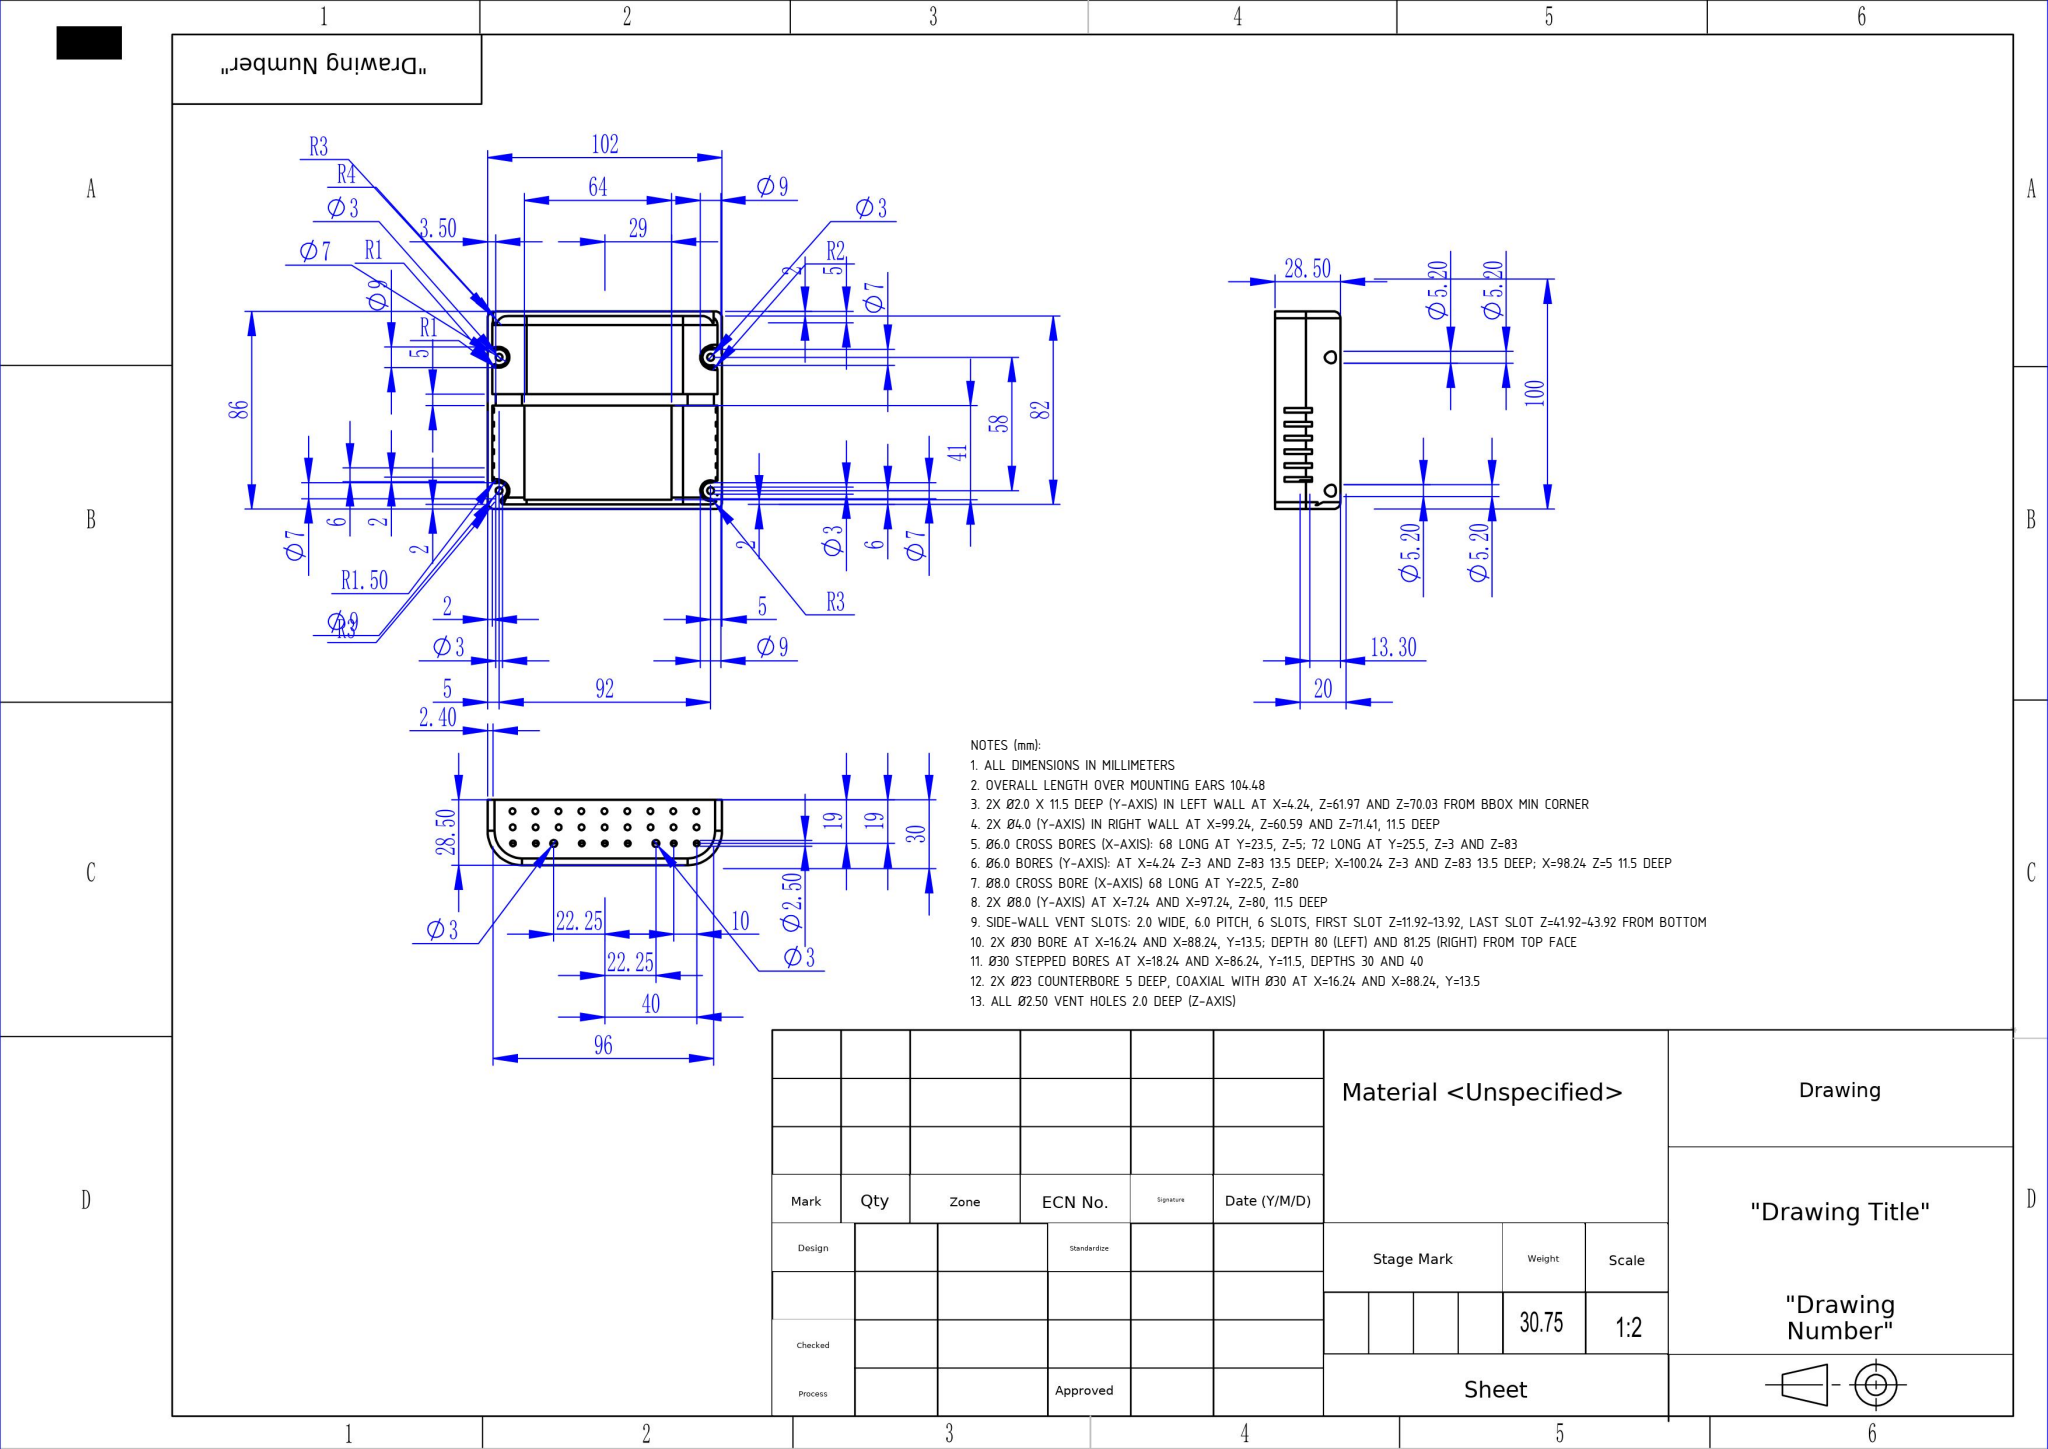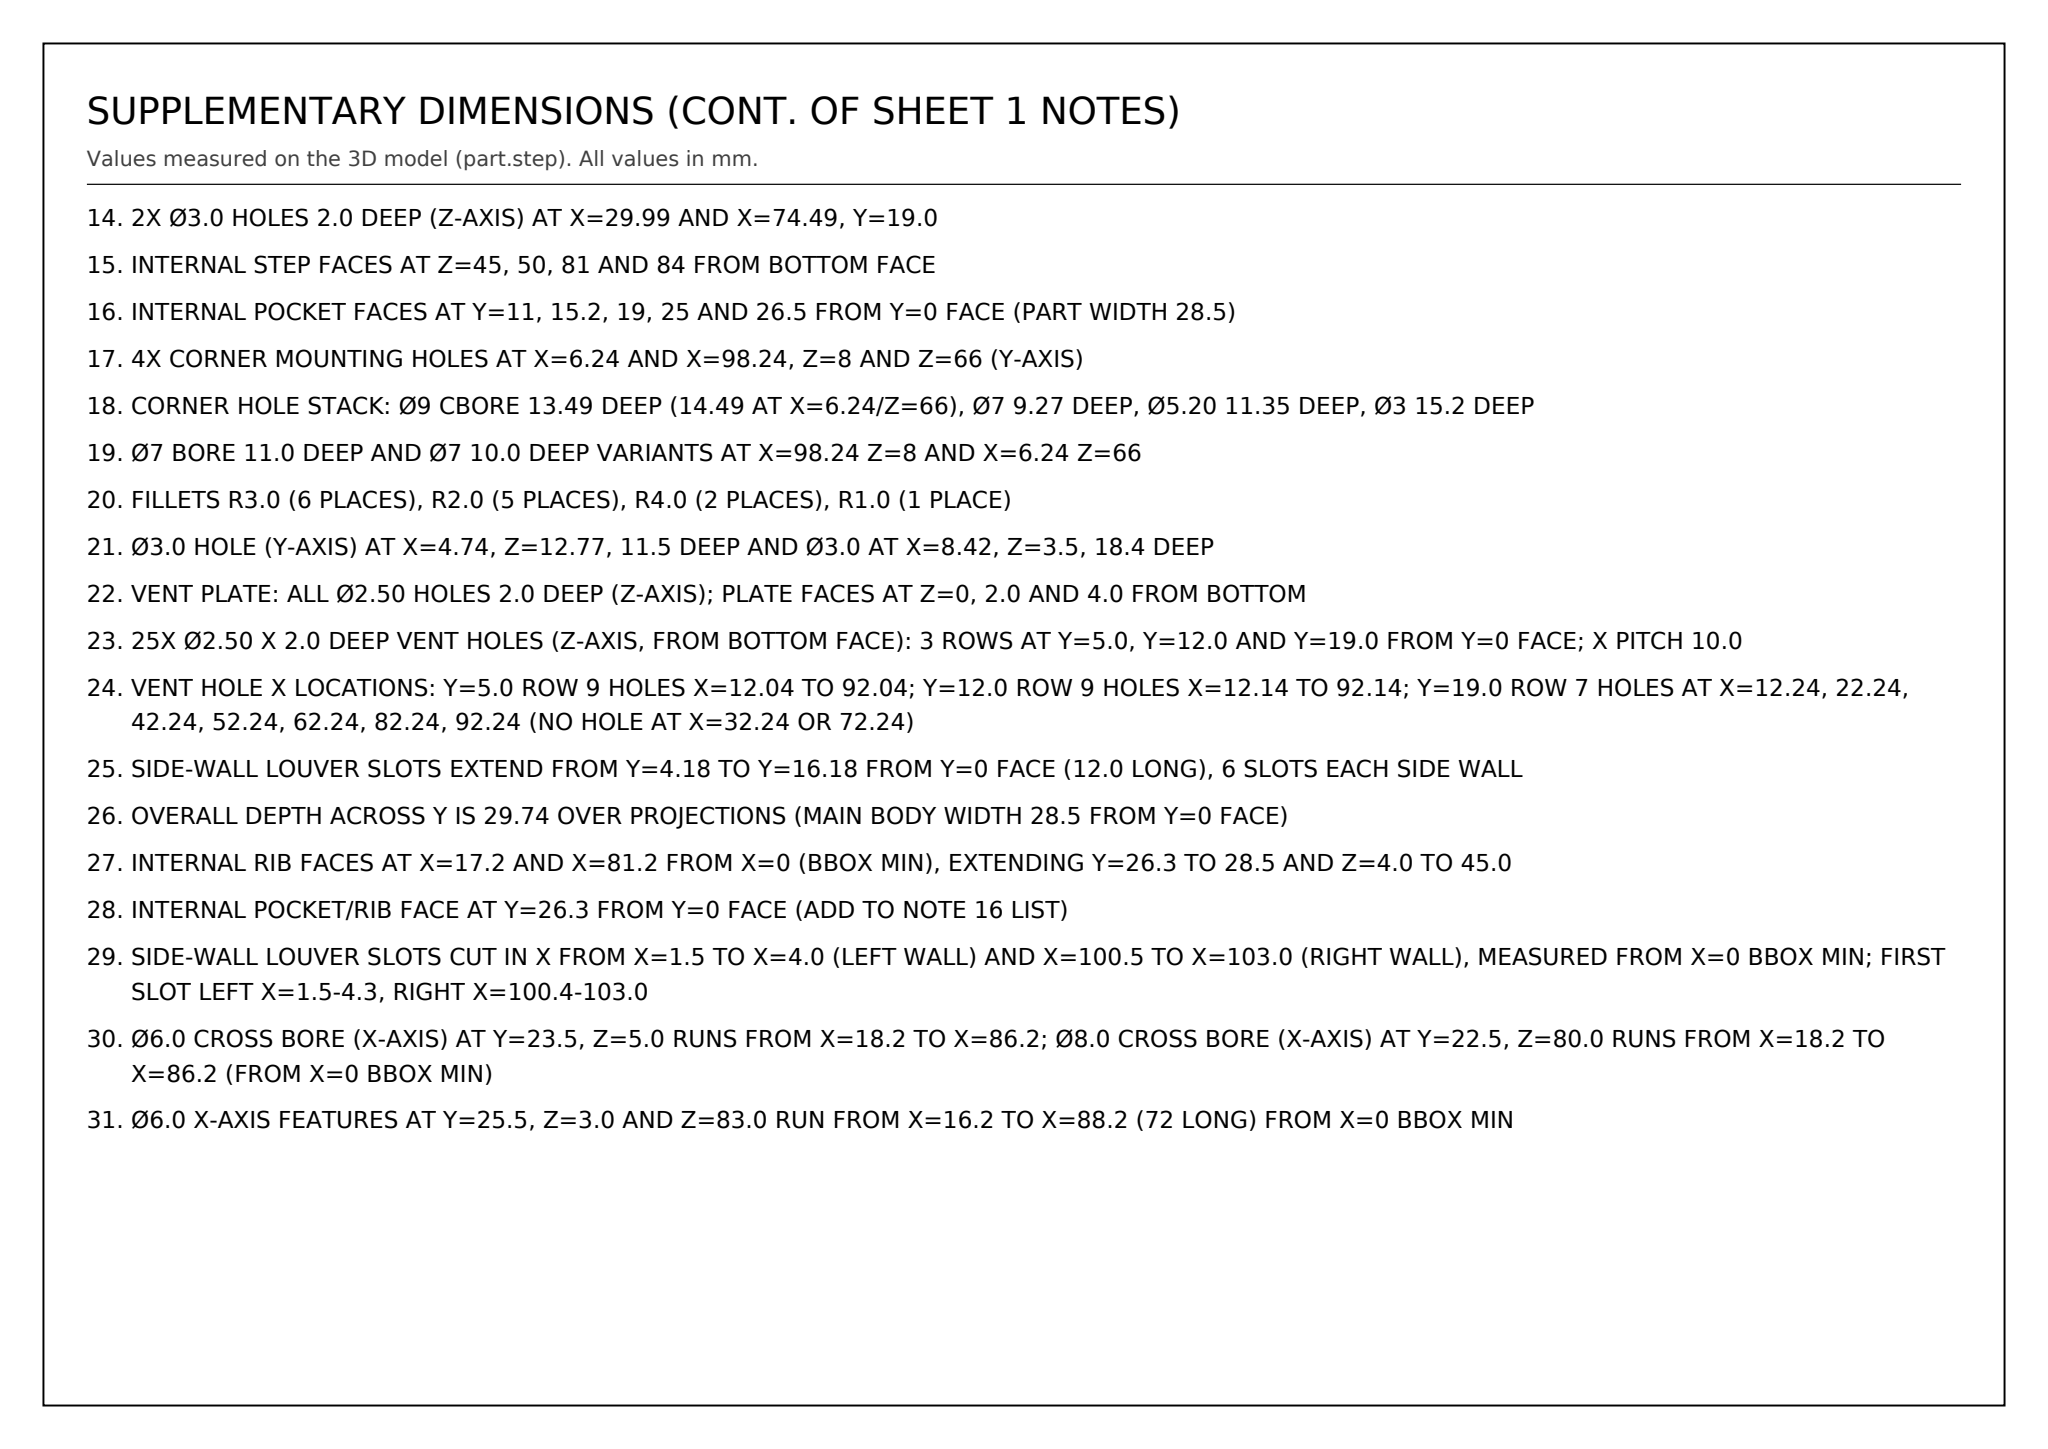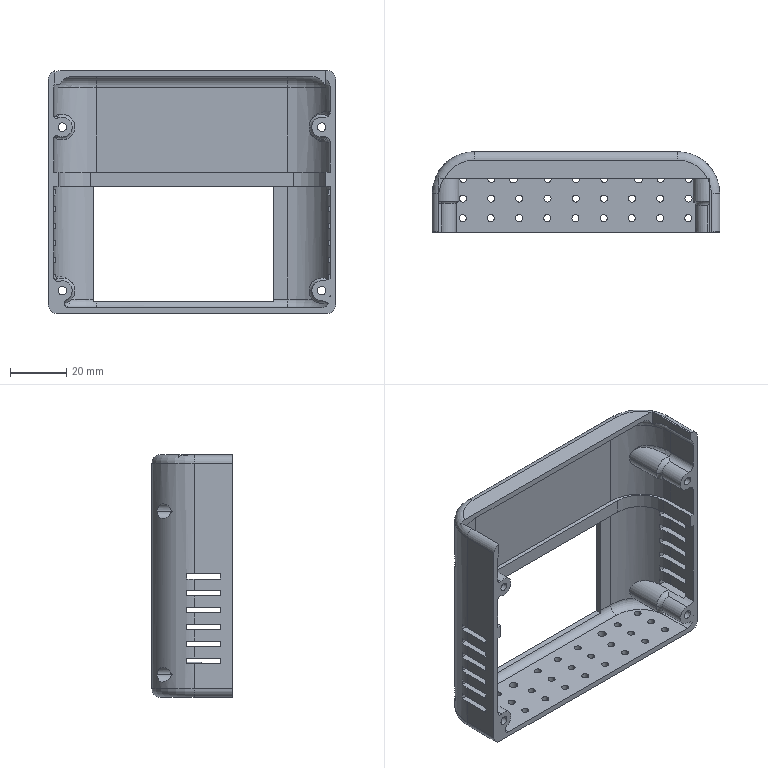Part | SolidWorks | mm | 1 solid | 221 faces | box 102 x 28.5 x 86 mm | volume 30750 mm3 | cylinder 108 | plane 86 | torus 14 | spline 11 | sphere 2 | commonest cylinder face diameters 2.5 x50 3 x14 5.2 x8 6 x8 7 x7 9 x6 30 x6 8 x3
Drawing notes:
ALL DIMENSIONS IN MILLIMETERS | from the solid: STEP facts header: units mm
OVERALL LENGTH OVER MOUNTING EARS 104.48 | from the solid: bbox_xyz x = 104.478
2X Ø2.0 X 11.5 DEEP (Y-AXIS) IN LEFT WALL AT X=4.24, Z=61.97 AND Z=70.03 FROM BBOX MIN CORNER | from the solid: Ø2.0 y-axis cylinders at (x=4.2, z=62.0) and (x=4.2, z=70.0), from y=0.0 to y=11.5 (blind, not through part width 28.5/29.74)
2X Ø4.0 (Y-AXIS) IN RIGHT WALL AT X=99.24, Z=60.59 AND Z=71.41, 11.5 DEEP | from the solid: cylinders 4.0 y [99.24,null,60.59] and [99.24,null,71.41] length 11.5
Ø6.0 CROSS BORES (X-AXIS): 68 LONG AT Y=23.5, Z=5; 72 LONG AT Y=25.5, Z=3 AND Z=83 | from the solid: cylinders 6.0 x [null,23.5,5] L68; [null,25.5,3] L72; [null,25.5,83] L72
Ø6.0 BORES (Y-AXIS): AT X=4.24 Z=3 AND Z=83 13.5 DEEP; X=100.24 Z=3 AND Z=83 13.5 DEEP; X=98.24 Z=5 11.5 DEEP | from the solid: cylinders 6.0 y [4.24,...,3]/[4.24,...,83] L13.5; [100.24,...,3]/[100.24,...,83] L13.5; [98.24,...,5] L11.5
Ø8.0 CROSS BORE (X-AXIS) 68 LONG AT Y=22.5, Z=80 | from the solid: cylinders 8.0 x [null,22.5,80] length 68
2X Ø8.0 (Y-AXIS) AT X=7.24 AND X=97.24, Z=80, 11.5 DEEP | from the solid: cylinders 8.0 y [7.24,null,80] and [97.24,null,80] length 11.5
SIDE-WALL VENT SLOTS: 2.0 WIDE, 6.0 PITCH, 6 SLOTS, FIRST SLOT Z=11.92-13.92, LAST SLOT Z=41.92-43.92 FROM BOTTOM | from the solid: axis_planes z pairs 11.92/13.92, 17.92/19.92, 23.92/25.92, 29.92/31.92, 35.92/37.92, 41.92/43.92
2X Ø30 BORE AT X=16.24 AND X=88.24, Y=13.5; DEPTH 80 (LEFT) AND 81.25 (RIGHT) FROM TOP FACE | from the solid: cylinders 30.0 z [16.24,13.5] L80 and [88.24,13.5] L81.25
Ø30 STEPPED BORES AT X=18.24 AND X=86.24, Y=11.5, DEPTHS 30 AND 40 | from the solid: cylinders 30.0 z [18.24,11.5] L30 & L40; [86.24,11.5] L30 & L40
2X Ø23 COUNTERBORE 5 DEEP, COAXIAL WITH Ø30 AT X=16.24 AND X=88.24, Y=13.5 | from the solid: cylinders 23.0 z [16.24,13.5] L5 and [88.24,13.5] L5
ALL Ø2.50 VENT HOLES 2.0 DEEP (Z-AXIS) | from the solid: cylinders 2.5 z length 2.0 (all instances)
2X Ø3.0 HOLES 2.0 DEEP (Z-AXIS) AT X=29.99 AND X=74.49, Y=19.0 | from the solid: cylinders 3.0 z [29.99,19.0] and [74.49,19.0] length 2.0
INTERNAL STEP FACES AT Z=45, 50, 81 AND 84 FROM BOTTOM FACE | from the solid: axis_planes z offsets 45.0, 50.0, 81.0, 84.0
INTERNAL POCKET FACES AT Y=11, 15.2, 19, 25 AND 26.5 FROM Y=0 FACE (PART WIDTH 28.5) | from the solid: axis_planes y offsets 11.0, 15.2, 19.0, 25.0, 26.5, 28.5
4X CORNER MOUNTING HOLES AT X=6.24 AND X=98.24, Z=8 AND Z=66 (Y-AXIS) | from the solid: cylinders 5.2 y [6.24,null,8], [6.24,null,66], [98.24,null,8], [98.24,null,66]
CORNER HOLE STACK: Ø9 CBORE 13.49 DEEP (14.49 AT X=6.24/Z=66), Ø7 9.27 DEEP, Ø5.20 11.35 DEEP, Ø3 15.2 DEEP | from the solid: cylinders 9.0 y L13.49/14.49; 7.0 y L9.27; 5.2 y L11.35; 3.0 y [6.24/98.24,...,8/66] L15.2
Ø7 BORE 11.0 DEEP AND Ø7 10.0 DEEP VARIANTS AT X=98.24 Z=8 AND X=6.24 Z=66 | from the solid: cylinders 7.0 y [98.24,null,8] L11.0; [6.24,null,66] L10.0
FILLETS R3.0 (6 PLACES), R2.0 (5 PLACES), R4.0 (2 PLACES), R1.0 (1 PLACE) | from the solid: fillet_radii [[2.0,5],[4.0,2],[3.0,6],[1.0,1]]
Ø3.0 HOLE (Y-AXIS) AT X=4.74, Z=12.77, 11.5 DEEP AND Ø3.0 AT X=8.42, Z=3.5, 18.4 DEEP | from the solid: cylinders 3.0 y [4.74,null,12.77] L11.5; [8.42,null,3.5] L18.4
VENT PLATE: ALL Ø2.50 HOLES 2.0 DEEP (Z-AXIS); PLATE FACES AT Z=0, 2.0 AND 4.0 FROM BOTTOM | from the solid: cylinders dia 2.5 axis z length 2.0; axis_planes z = 0.0, 2.0, 4.0
25X Ø2.50 X 2.0 DEEP VENT HOLES (Z-AXIS, FROM BOTTOM FACE): 3 ROWS AT Y=5.0, Y=12.0 AND Y=19.0 FROM Y=0 FACE; X PITCH 10.0 | from the solid: cylinders dia 2.5 axis z at y=5.0, 12.0, 19.0, length 2.0
VENT HOLE X LOCATIONS: Y=5.0 ROW 9 HOLES X=12.04 TO 92.04; Y=12.0 ROW 9 HOLES X=12.14 TO 92.14; Y=19.0 ROW 7 HOLES AT X=12.24, 22.24, 42.24, 52.24, 62.24, 82.24, 92.24 (NO HOLE AT X=32.24 OR 72.24) | from the solid: cylinders dia 2.5 axis z pos list (12.04...92.04 / 12.14...92.14 / 12.24...92.24)
SIDE-WALL LOUVER SLOTS EXTEND FROM Y=4.18 TO Y=16.18 FROM Y=0 FACE (12.0 LONG), 6 SLOTS EACH SIDE WALL | from the solid: axis_planes y=4.18 (12 faces) and y=16.18 (12 faces)
OVERALL DEPTH ACROSS Y IS 29.74 OVER PROJECTIONS (MAIN BODY WIDTH 28.5 FROM Y=0 FACE) | from the solid: bbox_xyz y = 29.742; axis_plane y=28.5
INTERNAL RIB FACES AT X=17.2 AND X=81.2 FROM X=0 (BBOX MIN), EXTENDING Y=26.3 TO 28.5 AND Z=4.0 TO 45.0 | from the solid: axis_planes normal x offset 17.2 and 81.2, extent y[26.3,28.5] z[4.0,45.0]
INTERNAL POCKET/RIB FACE AT Y=26.3 FROM Y=0 FACE (ADD TO NOTE 16 LIST) | from the solid: axis_planes x=17.2 / x=81.2 extent y starts at 26.3
SIDE-WALL LOUVER SLOTS CUT IN X FROM X=1.5 TO X=4.0 (LEFT WALL) AND X=100.5 TO X=103.0 (RIGHT WALL), MEASURED FROM X=0 BBOX MIN; FIRST SLOT LEFT X=1.5-4.3, RIGHT X=100.4-103.0 | from the solid: axis_planes normal y offset 16.2, extents x[1.5,4.0]/[1.5,4.3] and x[100.5,103.0]/[100.4,103.0]
Ø6.0 CROSS BORE (X-AXIS) AT Y=23.5, Z=5.0 RUNS FROM X=18.2 TO X=86.2; Ø8.0 CROSS BORE (X-AXIS) AT Y=22.5, Z=80.0 RUNS FROM X=18.2 TO X=86.2 (FROM X=0 BBOX MIN) | from the solid: concave arcs dia 6.0 x-axis y23.5 z5.0 from 18.2 to 86.2; dia 8.0 x-axis y22.5 z80.0 from 18.2 to 86.2
Ø6.0 X-AXIS FEATURES AT Y=25.5, Z=3.0 AND Z=83.0 RUN FROM X=16.2 TO X=88.2 (72 LONG) FROM X=0 BBOX MIN | from the solid: convex arcs dia 6.0 x-axis y25.5 z3.0 and z83.0 from 16.2 to 88.2